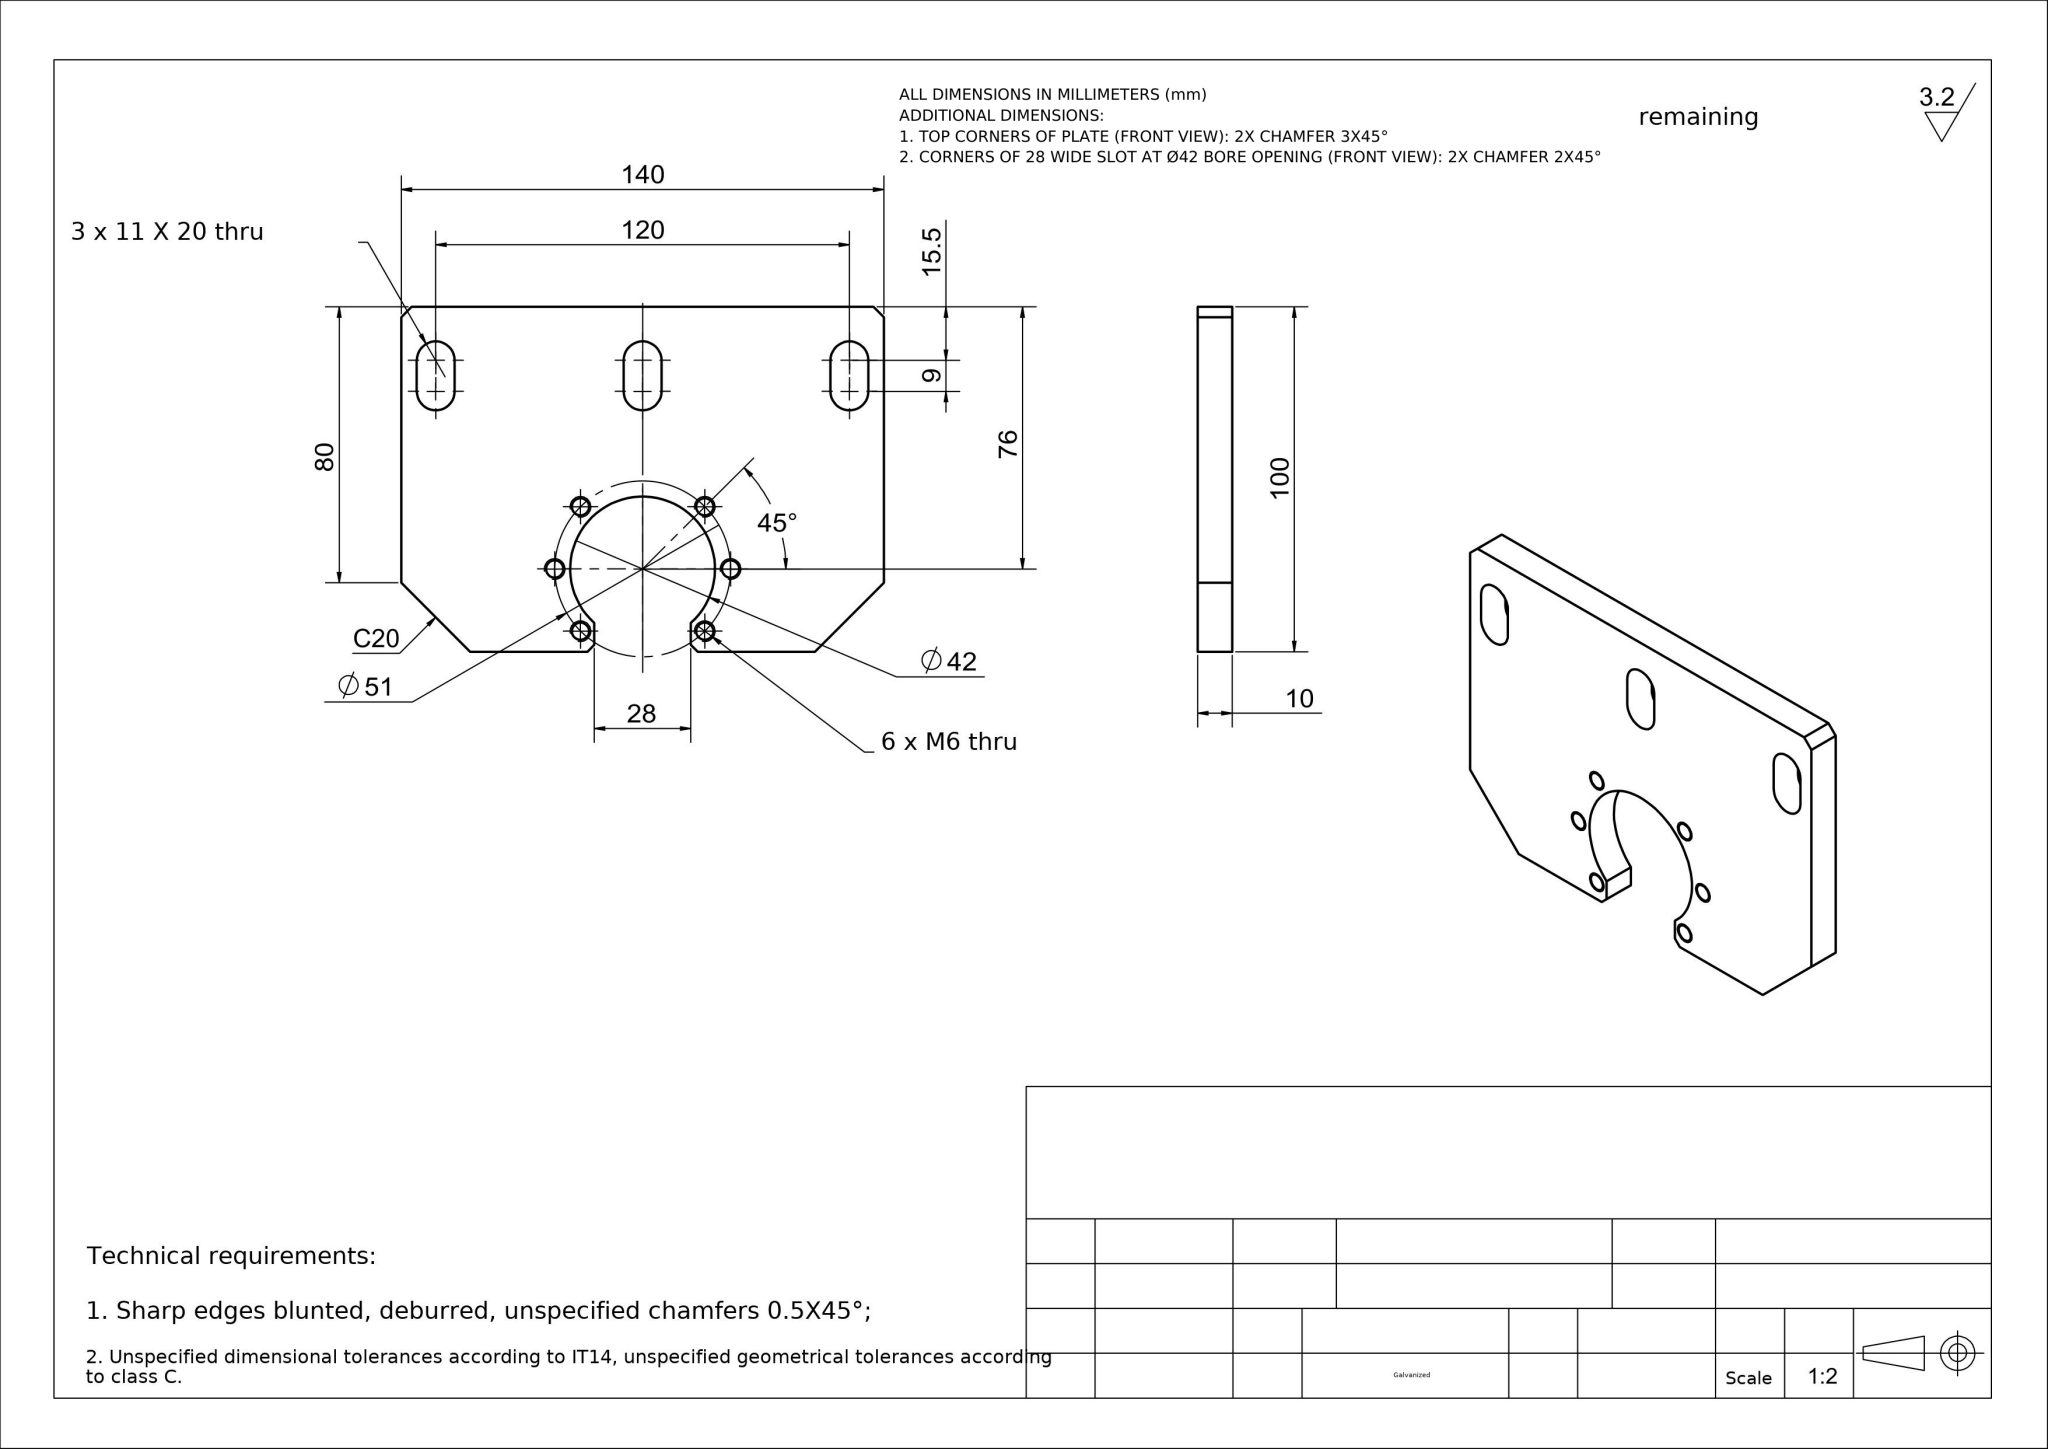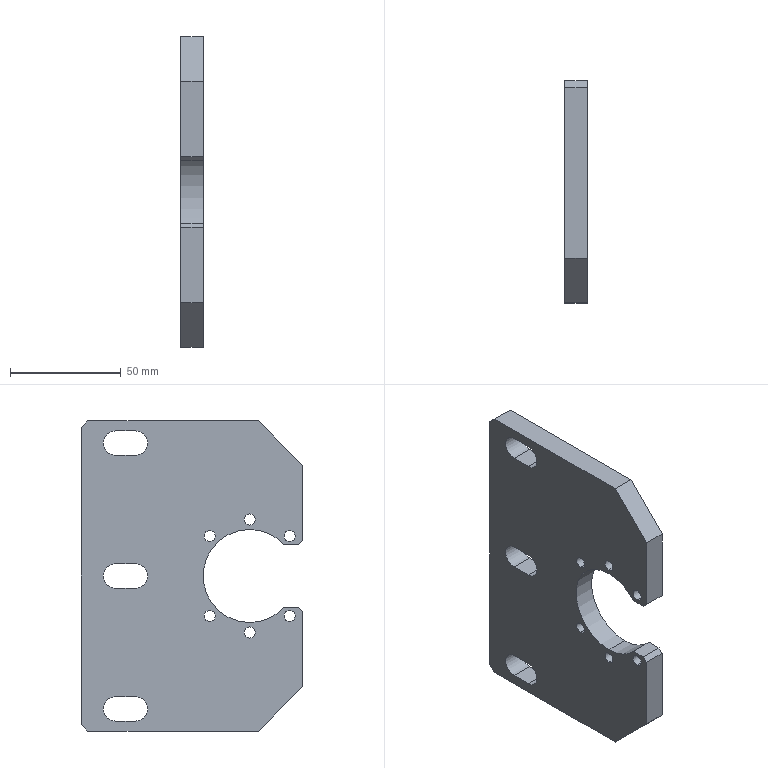Part | NX | mm | 1 solid | 42 faces | box 10 x 100 x 140 mm | volume 113706 mm3 | cylinder 21 | plane 21 | commonest cylinder face diameters 5 x12 11 x6 42 x3